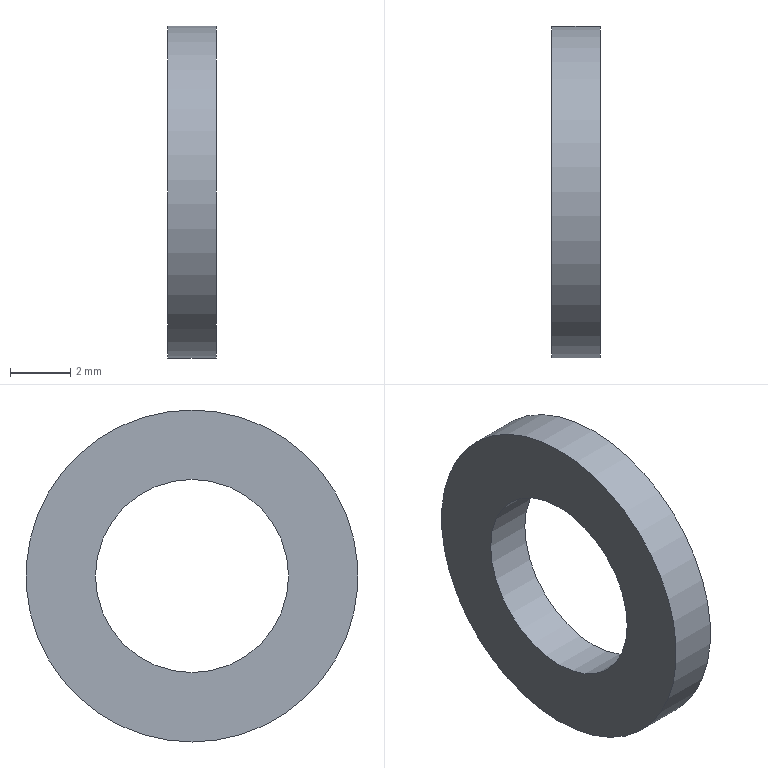Component | NX | GB-T848-2002_M6_2 | 1 solid | 4 faces | box 1.6 x 11 x 11 mm | volume 101 mm3 | cylinder 2 | plane 2 | commonest cylinder face diameters 11 x1 6.4 x1
STEP:
#1=CARTESIAN_POINT('',(0.,0.,0.));
#2=DIRECTION('',(0.,0.,1.));
#3=DIRECTION('',(1.,0.,0.));
#4=AXIS2_PLACEMENT_3D('',#1,#2,#3);
#5=CARTESIAN_POINT('',(13.6,32.,-62.5));
#6=VERTEX_POINT('',#5);
#7=CARTESIAN_POINT('',(13.6,32.,-57.));
#8=DIRECTION('',(1.,0.,0.));
#9=DIRECTION('',(0.,0.,-1.));
#10=AXIS2_PLACEMENT_3D('',#7,#8,#9);
#11=CIRCLE('',#10,5.5);
#12=CARTESIAN_POINT('',(13.6,32.,-57.));
#13=DIRECTION('',(-1.,0.,0.));
#14=DIRECTION('',(0.,0.,1.));
#15=AXIS2_PLACEMENT_3D('',#12,#13,#14);
#16=CYLINDRICAL_SURFACE('',#15,5.5);
#17=CARTESIAN_POINT('',(9.425,0.));
#18=DIRECTION('',(-1.,0.));
#19=VECTOR('',#18,1.);
#20=LINE('',#17,#19);
#21=(GEOMETRIC_REPRESENTATION_CONTEXT(2)PARAMETRIC_REPRESENTATION_CONTEXT()REPRESENTATION_CONTEXT('',''));
#22=DEFINITIONAL_REPRESENTATION('',(#20),#21);
#23=PCURVE('',#16,#22);
#24=CARTESIAN_POINT('',(13.6,32.,-57.));
#25=DIRECTION('',(1.,0.,0.));
#26=DIRECTION('',(0.,0.,-1.));
#27=AXIS2_PLACEMENT_3D('',#24,#25,#26);
#28=PLANE('',#27);
#29=CARTESIAN_POINT('',(0.,0.));
#30=DIRECTION('',(1.,0.));
#31=AXIS2_PLACEMENT_2D('',#29,#30);
#32=CIRCLE('',#31,5.5);
#33=(GEOMETRIC_REPRESENTATION_CONTEXT(2)PARAMETRIC_REPRESENTATION_CONTEXT()REPRESENTATION_CONTEXT('',''));
#34=DEFINITIONAL_REPRESENTATION('',(#32),#33);
#35=PCURVE('',#28,#34);
#36=SURFACE_CURVE('',#11,(#23,#35),.PCURVE_S1.);
#37=EDGE_CURVE('',#6,#6,#36,.T.);
#38=ORIENTED_EDGE('',*,*,#37,.F.);
#39=CARTESIAN_POINT('',(12.,32.,-62.5));
#40=VERTEX_POINT('',#39);
#41=CARTESIAN_POINT('',(13.6,32.,-62.5));
#42=CARTESIAN_POINT('',(12.,32.,-62.5));
#43=B_SPLINE_CURVE_WITH_KNOTS('',1,(#41,#42),.UNSPECIFIED.,.F.,.F.,(2,2),(0.,1.6),.PIECEWISE_BEZIER_KNOTS.);
#44=CARTESIAN_POINT('',(9.425,0.));
#45=DIRECTION('',(0.,1.));
#46=VECTOR('',#45,1.);
#47=LINE('',#44,#46);
#48=(GEOMETRIC_REPRESENTATION_CONTEXT(2)PARAMETRIC_REPRESENTATION_CONTEXT()REPRESENTATION_CONTEXT('',''));
#49=DEFINITIONAL_REPRESENTATION('',(#47),#48);
#50=PCURVE('',#16,#49);
#51=CARTESIAN_POINT('',(3.142,0.));
#52=DIRECTION('',(0.,1.));
#53=VECTOR('',#52,1.);
#54=LINE('',#51,#53);
#55=(GEOMETRIC_REPRESENTATION_CONTEXT(2)PARAMETRIC_REPRESENTATION_CONTEXT()REPRESENTATION_CONTEXT('',''));
#56=DEFINITIONAL_REPRESENTATION('',(#54),#55);
#57=PCURVE('',#16,#56);
#58=SEAM_CURVE('',#43,(#50,#57),.PCURVE_S1.);
#59=EDGE_CURVE('',#6,#40,#58,.T.);
#60=ORIENTED_EDGE('',*,*,#59,.T.);
#61=CARTESIAN_POINT('',(12.,32.,-57.));
#62=DIRECTION('',(1.,0.,0.));
#63=DIRECTION('',(0.,0.,-1.));
#64=AXIS2_PLACEMENT_3D('',#61,#62,#63);
#65=CIRCLE('',#64,5.5);
#66=CARTESIAN_POINT('',(9.425,1.6));
#67=DIRECTION('',(-1.,0.));
#68=VECTOR('',#67,1.);
#69=LINE('',#66,#68);
#70=(GEOMETRIC_REPRESENTATION_CONTEXT(2)PARAMETRIC_REPRESENTATION_CONTEXT()REPRESENTATION_CONTEXT('',''));
#71=DEFINITIONAL_REPRESENTATION('',(#69),#70);
#72=PCURVE('',#16,#71);
#73=CARTESIAN_POINT('',(12.,32.,-57.));
#74=DIRECTION('',(1.,0.,0.));
#75=DIRECTION('',(0.,0.,-1.));
#76=AXIS2_PLACEMENT_3D('',#73,#74,#75);
#77=PLANE('',#76);
#78=CARTESIAN_POINT('',(0.,0.));
#79=DIRECTION('',(1.,0.));
#80=AXIS2_PLACEMENT_2D('',#78,#79);
#81=CIRCLE('',#80,5.5);
#82=(GEOMETRIC_REPRESENTATION_CONTEXT(2)PARAMETRIC_REPRESENTATION_CONTEXT()REPRESENTATION_CONTEXT('',''));
#83=DEFINITIONAL_REPRESENTATION('',(#81),#82);
#84=PCURVE('',#77,#83);
#85=SURFACE_CURVE('',#65,(#72,#84),.PCURVE_S1.);
#86=EDGE_CURVE('',#40,#40,#85,.T.);
#87=ORIENTED_EDGE('',*,*,#86,.T.);
#88=ORIENTED_EDGE('',*,*,#59,.F.);
#89=EDGE_LOOP('',(#38,#60,#87,#88));
#90=FACE_BOUND('',#89,.T.);
#91=ADVANCED_FACE('',(#90),#16,.T.);
#92=CARTESIAN_POINT('',(13.6,32.,-60.2));
#93=VERTEX_POINT('',#92);
#94=CARTESIAN_POINT('',(13.6,32.,-57.));
#95=DIRECTION('',(1.,0.,0.));
#96=DIRECTION('',(0.,0.,-1.));
#97=AXIS2_PLACEMENT_3D('',#94,#95,#96);
#98=CIRCLE('',#97,3.2);
#99=CARTESIAN_POINT('',(13.6,32.,-57.));
#100=DIRECTION('',(-1.,0.,0.));
#101=DIRECTION('',(0.,0.,1.));
#102=AXIS2_PLACEMENT_3D('',#99,#100,#101);
#103=CYLINDRICAL_SURFACE('',#102,3.2);
#104=CARTESIAN_POINT('',(9.425,0.));
#105=DIRECTION('',(-1.,0.));
#106=VECTOR('',#105,1.);
#107=LINE('',#104,#106);
#108=(GEOMETRIC_REPRESENTATION_CONTEXT(2)PARAMETRIC_REPRESENTATION_CONTEXT()REPRESENTATION_CONTEXT('',''));
#109=DEFINITIONAL_REPRESENTATION('',(#107),#108);
#110=PCURVE('',#103,#109);
#111=CARTESIAN_POINT('',(0.,0.));
#112=DIRECTION('',(1.,0.));
#113=AXIS2_PLACEMENT_2D('',#111,#112);
#114=CIRCLE('',#113,3.2);
#115=(GEOMETRIC_REPRESENTATION_CONTEXT(2)PARAMETRIC_REPRESENTATION_CONTEXT()REPRESENTATION_CONTEXT('',''));
#116=DEFINITIONAL_REPRESENTATION('',(#114),#115);
#117=PCURVE('',#28,#116);
#118=SURFACE_CURVE('',#98,(#110,#117),.PCURVE_S1.);
#119=EDGE_CURVE('',#93,#93,#118,.T.);
#120=ORIENTED_EDGE('',*,*,#119,.F.);
#121=CARTESIAN_POINT('',(12.,32.,-60.2));
#122=VERTEX_POINT('',#121);
#123=CARTESIAN_POINT('',(13.6,32.,-60.2));
#124=CARTESIAN_POINT('',(12.,32.,-60.2));
#125=B_SPLINE_CURVE_WITH_KNOTS('',1,(#123,#124),.UNSPECIFIED.,.F.,.F.,(2,2),(0.,1.6),.PIECEWISE_BEZIER_KNOTS.);
#126=CARTESIAN_POINT('',(9.425,0.));
#127=DIRECTION('',(0.,1.));
#128=VECTOR('',#127,1.);
#129=LINE('',#126,#128);
#130=(GEOMETRIC_REPRESENTATION_CONTEXT(2)PARAMETRIC_REPRESENTATION_CONTEXT()REPRESENTATION_CONTEXT('',''));
#131=DEFINITIONAL_REPRESENTATION('',(#129),#130);
#132=PCURVE('',#103,#131);
#133=CARTESIAN_POINT('',(3.142,0.));
#134=DIRECTION('',(0.,1.));
#135=VECTOR('',#134,1.);
#136=LINE('',#133,#135);
#137=(GEOMETRIC_REPRESENTATION_CONTEXT(2)PARAMETRIC_REPRESENTATION_CONTEXT()REPRESENTATION_CONTEXT('',''));
#138=DEFINITIONAL_REPRESENTATION('',(#136),#137);
#139=PCURVE('',#103,#138);
#140=SEAM_CURVE('',#125,(#132,#139),.PCURVE_S1.);
#141=EDGE_CURVE('',#93,#122,#140,.T.);
#142=ORIENTED_EDGE('',*,*,#141,.T.);
#143=CARTESIAN_POINT('',(12.,32.,-57.));
#144=DIRECTION('',(1.,0.,0.));
#145=DIRECTION('',(0.,0.,-1.));
#146=AXIS2_PLACEMENT_3D('',#143,#144,#145);
#147=CIRCLE('',#146,3.2);
#148=CARTESIAN_POINT('',(9.425,1.6));
#149=DIRECTION('',(-1.,0.));
#150=VECTOR('',#149,1.);
#151=LINE('',#148,#150);
#152=(GEOMETRIC_REPRESENTATION_CONTEXT(2)PARAMETRIC_REPRESENTATION_CONTEXT()REPRESENTATION_CONTEXT('',''));
#153=DEFINITIONAL_REPRESENTATION('',(#151),#152);
#154=PCURVE('',#103,#153);
#155=CARTESIAN_POINT('',(0.,0.));
#156=DIRECTION('',(1.,0.));
#157=AXIS2_PLACEMENT_2D('',#155,#156);
#158=CIRCLE('',#157,3.2);
#159=(GEOMETRIC_REPRESENTATION_CONTEXT(2)PARAMETRIC_REPRESENTATION_CONTEXT()REPRESENTATION_CONTEXT('',''));
#160=DEFINITIONAL_REPRESENTATION('',(#158),#159);
#161=PCURVE('',#77,#160);
#162=SURFACE_CURVE('',#147,(#154,#161),.PCURVE_S1.);
#163=EDGE_CURVE('',#122,#122,#162,.T.);
#164=ORIENTED_EDGE('',*,*,#163,.T.);
#165=ORIENTED_EDGE('',*,*,#141,.F.);
#166=EDGE_LOOP('',(#120,#142,#164,#165));
#167=FACE_BOUND('',#166,.F.);
#168=ADVANCED_FACE('',(#167),#103,.F.);
#169=ORIENTED_EDGE('',*,*,#37,.T.);
#170=EDGE_LOOP('',(#169));
#171=FACE_BOUND('',#170,.T.);
#172=ORIENTED_EDGE('',*,*,#119,.F.);
#173=EDGE_LOOP('',(#172));
#174=FACE_BOUND('',#173,.T.);
#175=ADVANCED_FACE('',(#171,#174),#28,.T.);
#176=ORIENTED_EDGE('',*,*,#86,.F.);
#177=EDGE_LOOP('',(#176));
#178=FACE_BOUND('',#177,.T.);
#179=ORIENTED_EDGE('',*,*,#163,.T.);
#180=EDGE_LOOP('',(#179));
#181=FACE_BOUND('',#180,.T.);
#182=ADVANCED_FACE('',(#178,#181),#77,.F.);
#183=CLOSED_SHELL('',(#91,#168,#175,#182));
#184=MANIFOLD_SOLID_BREP('',#183);
#185=(LENGTH_UNIT()NAMED_UNIT(*)SI_UNIT(.MILLI.,.METRE.));
#186=UNCERTAINTY_MEASURE_WITH_UNIT(LENGTH_MEASURE(0.00001),#185,'','');
#187=(NAMED_UNIT(*)PLANE_ANGLE_UNIT()SI_UNIT($,.RADIAN.));
#188=(NAMED_UNIT(*)SI_UNIT($,.STERADIAN.)SOLID_ANGLE_UNIT());
#189=(GEOMETRIC_REPRESENTATION_CONTEXT(3)GLOBAL_UNCERTAINTY_ASSIGNED_CONTEXT((#186))GLOBAL_UNIT_ASSIGNED_CONTEXT((#185,#187,#188))REPRESENTATION_CONTEXT('',''));
#190=ADVANCED_BREP_SHAPE_REPRESENTATION('',(#4,#184),#189);